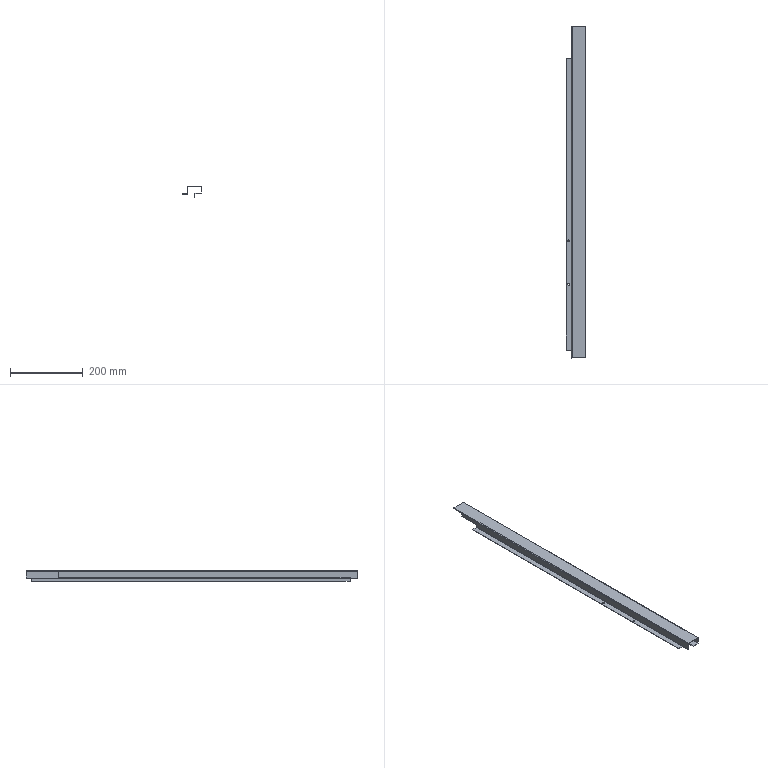Component | SolidWorks | CCQ-1.1-15LowerSidePost2-1 | 1 solid | 54 faces | volume 107225 mm3 | plane 40 | cylinder 14 | commonest cylinder face diameters 1.473 x5 3.473 x5 5 x4 | material 304